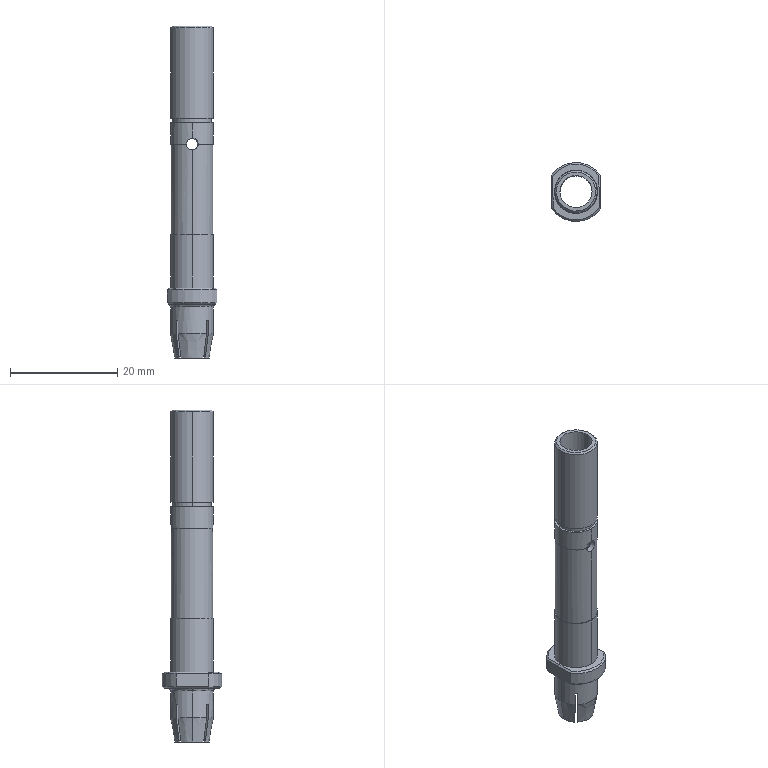Component | SolidWorks | MotorAssemblyWhen2-1_37bi-mpp70-3022-1 | 1 solid | 64 faces | volume 1337 mm3 | plane 31 | cylinder 20 | cone 11 | torus 2 | commonest cylinder face diameters 2.2 x4 8 x4 6 x2 7.9 x2 7.997 x2 7.8 x2 7.2 x2 11 x2